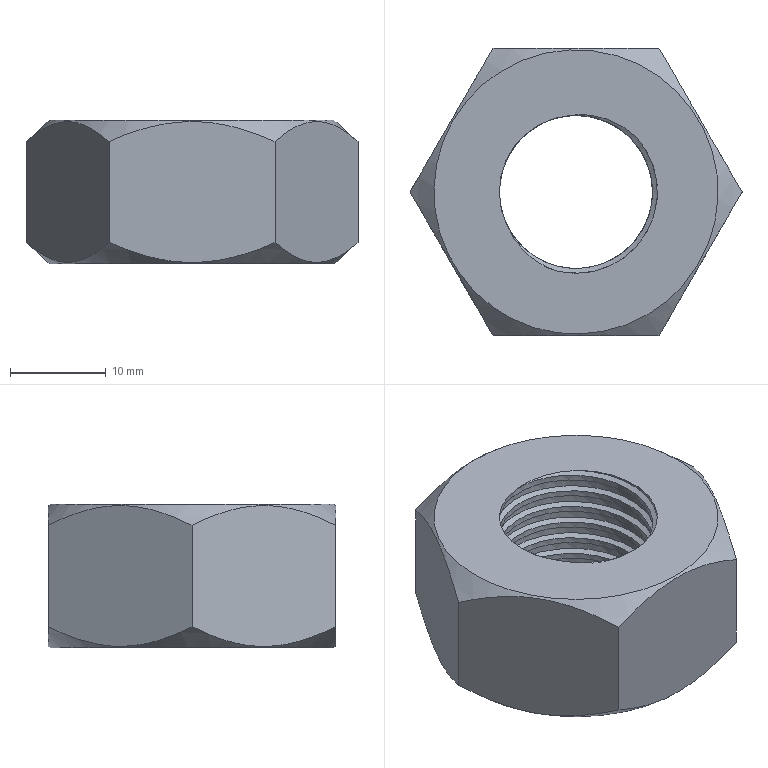Component | NX | 10__NUT_M16X1_5__2_2 | 1 solid | 15 faces | volume 8339 mm3 | plane 9 | cylinder 2 | cone 2 | spline 2 | commonest cylinder face diameters 16 x1 17 x1